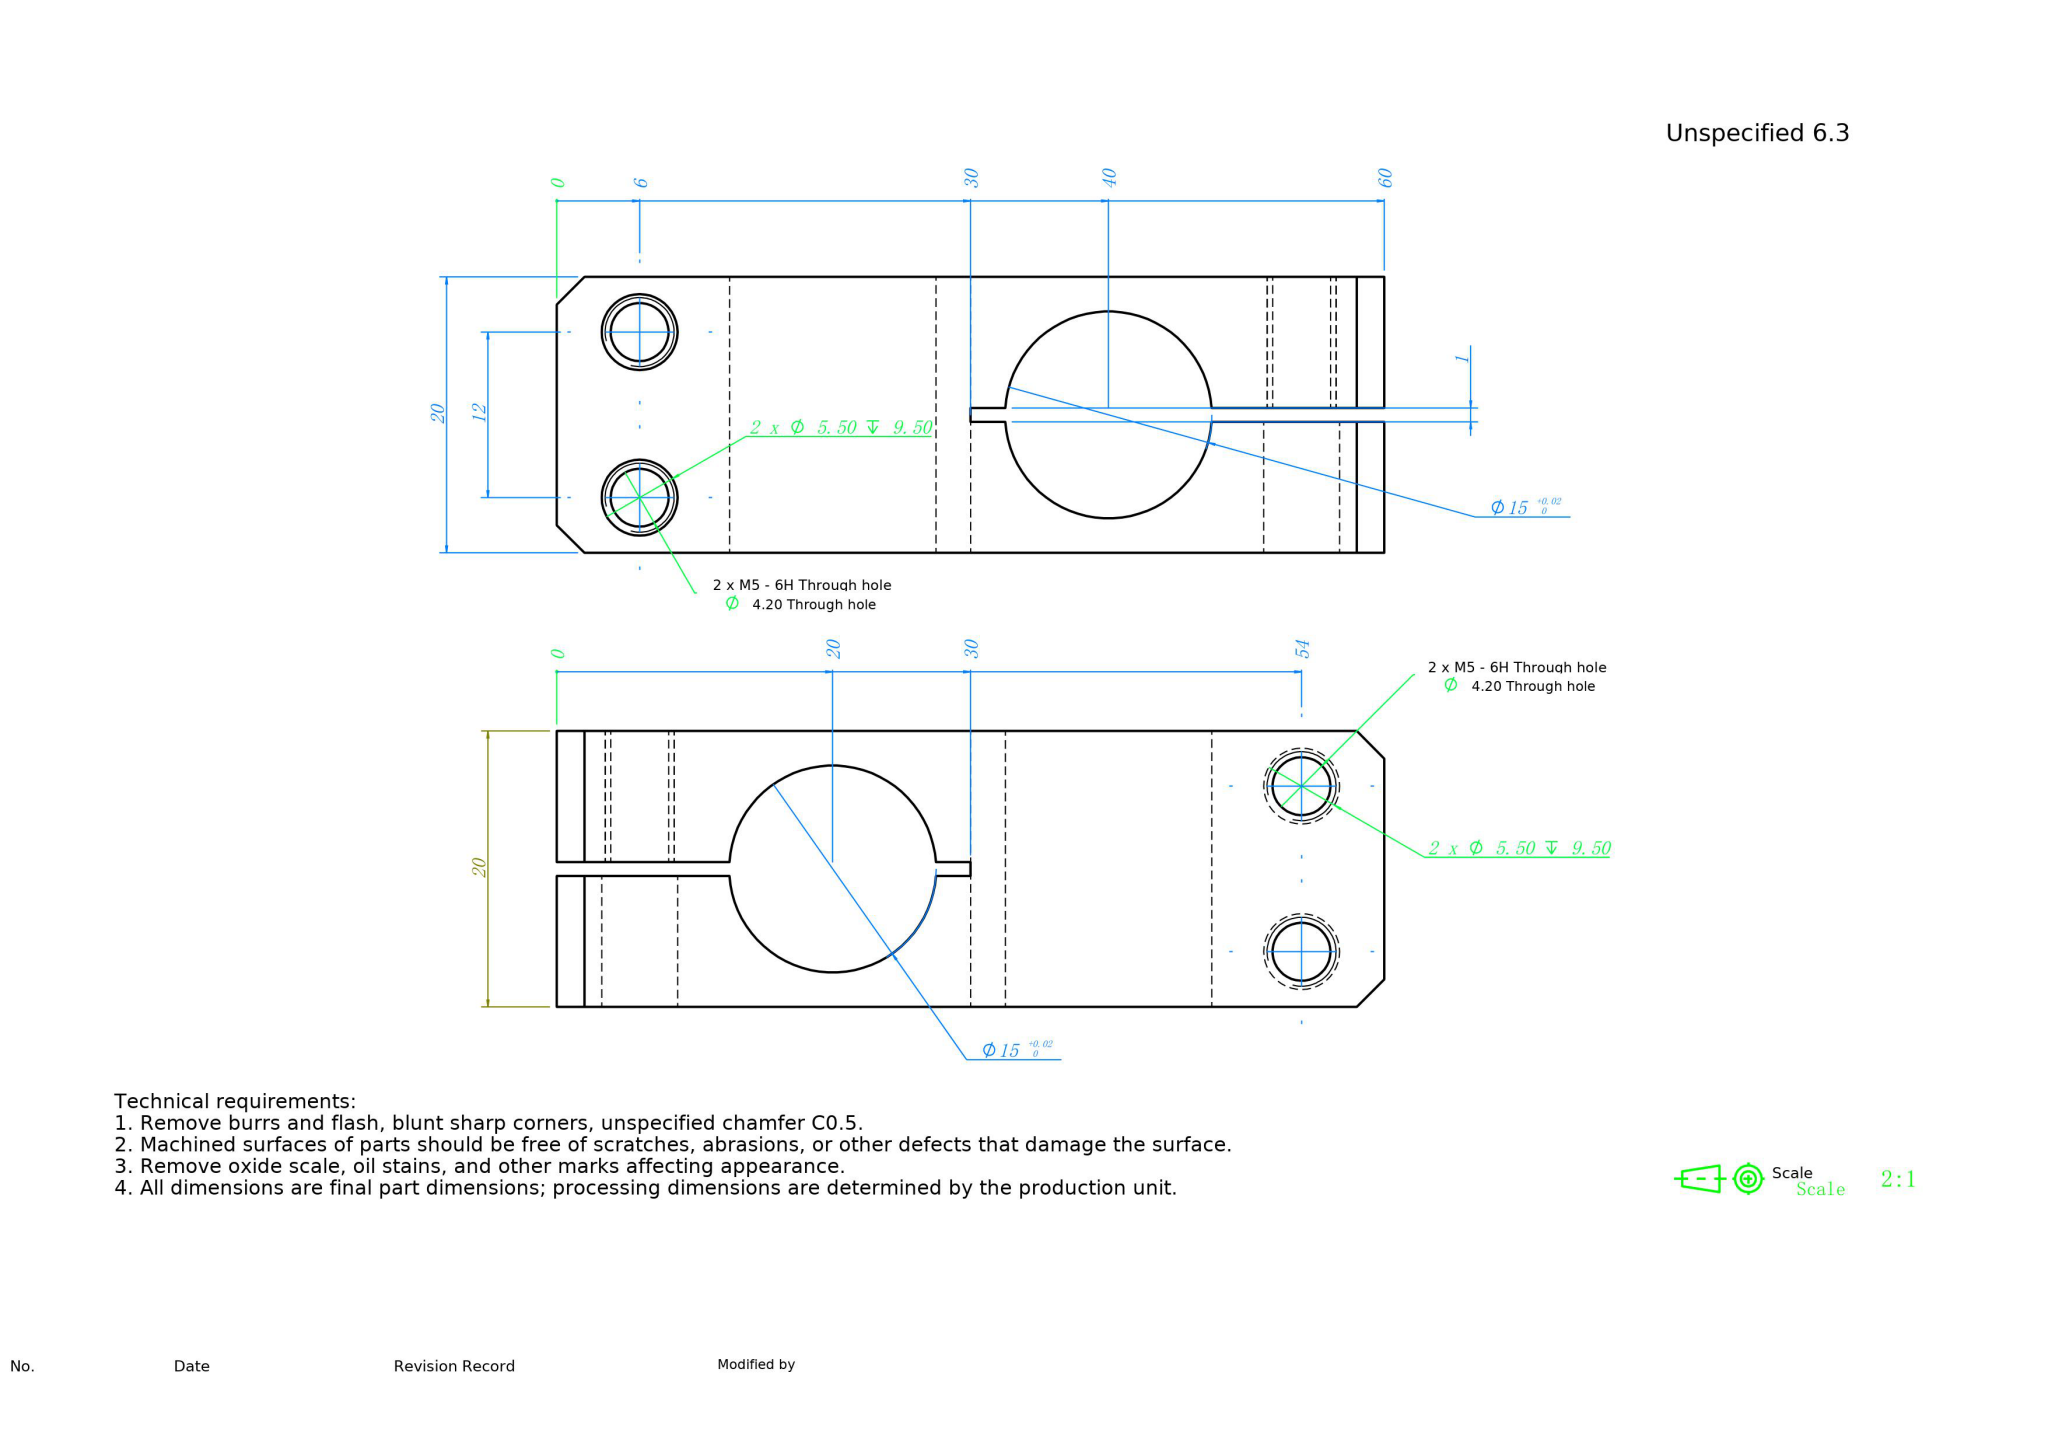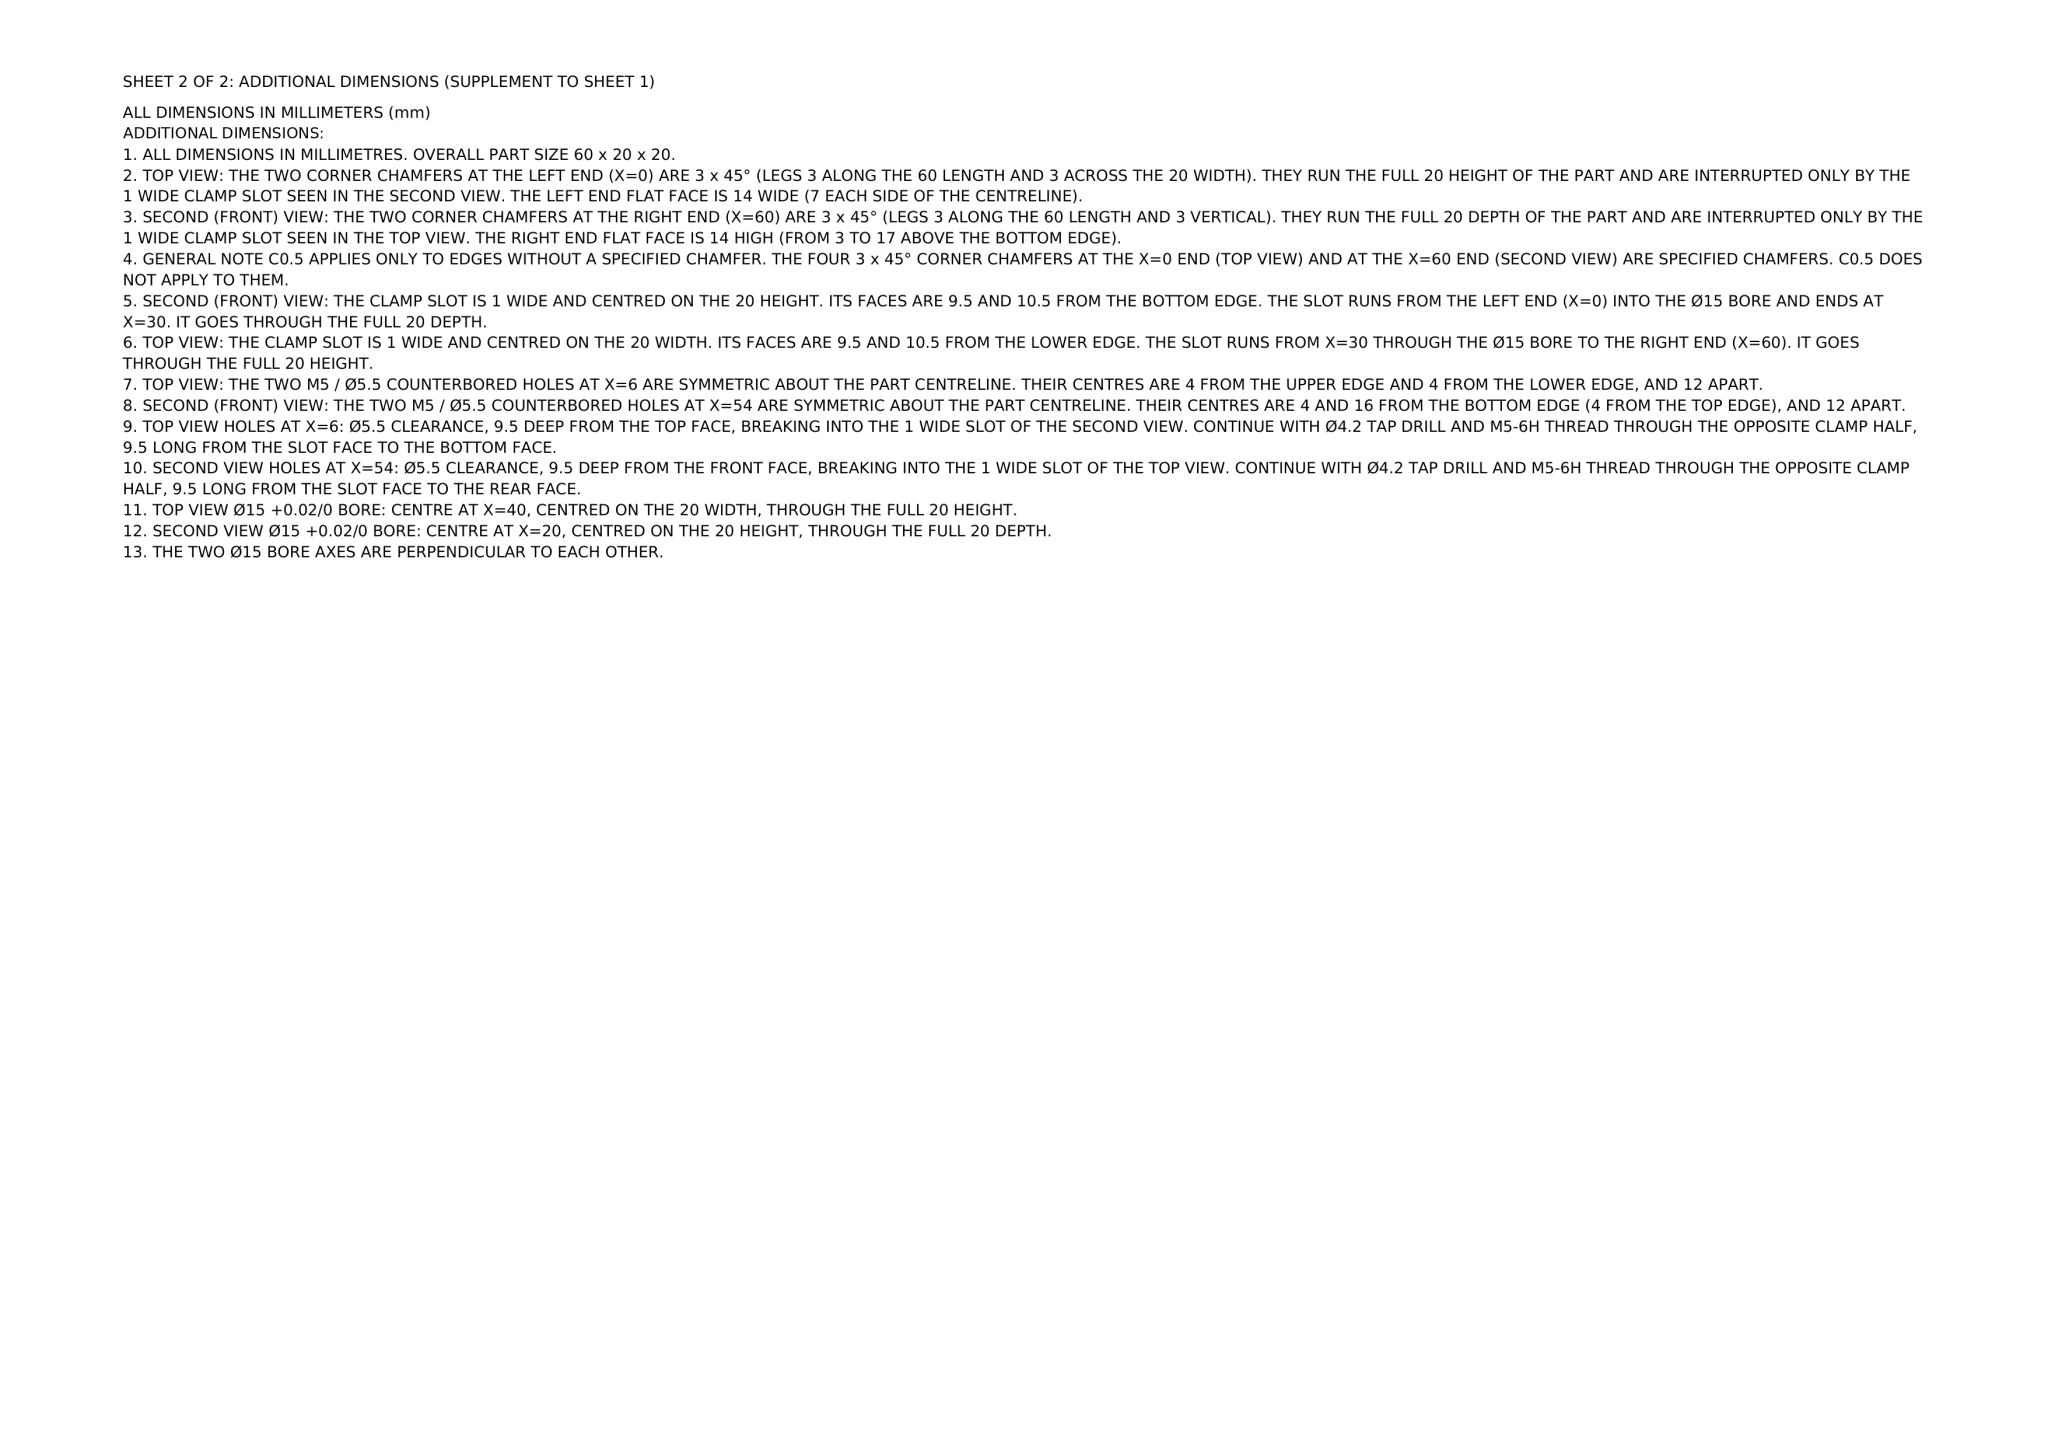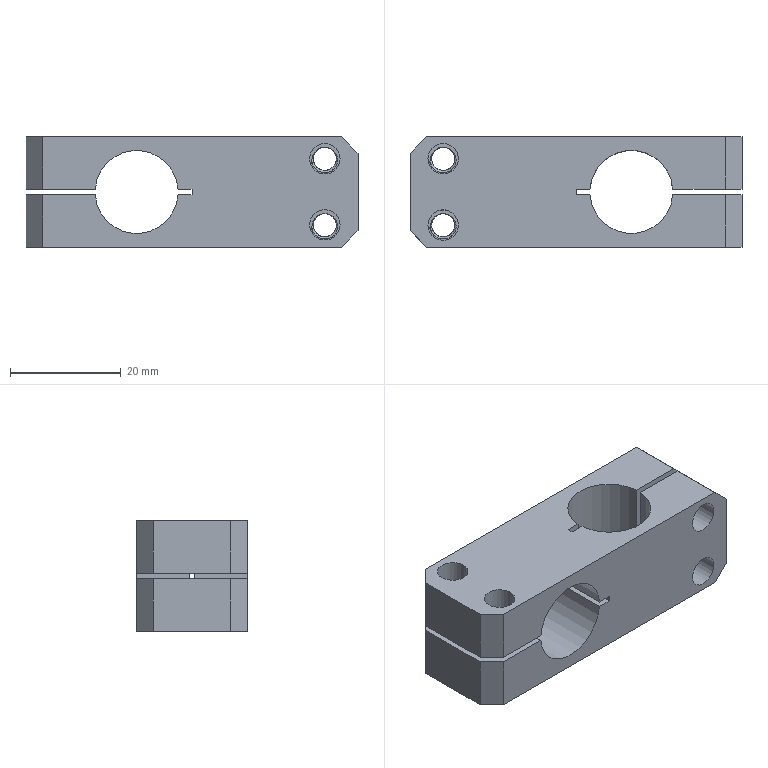Part | NX | mm | 1 solid | 52 faces | box 60 x 20 x 20 mm | volume 14444 mm3 | plane 28 | cylinder 16 | spline 8 | commonest cylinder face diameters 4.2 x4 5 x4 15 x4 5.5 x4